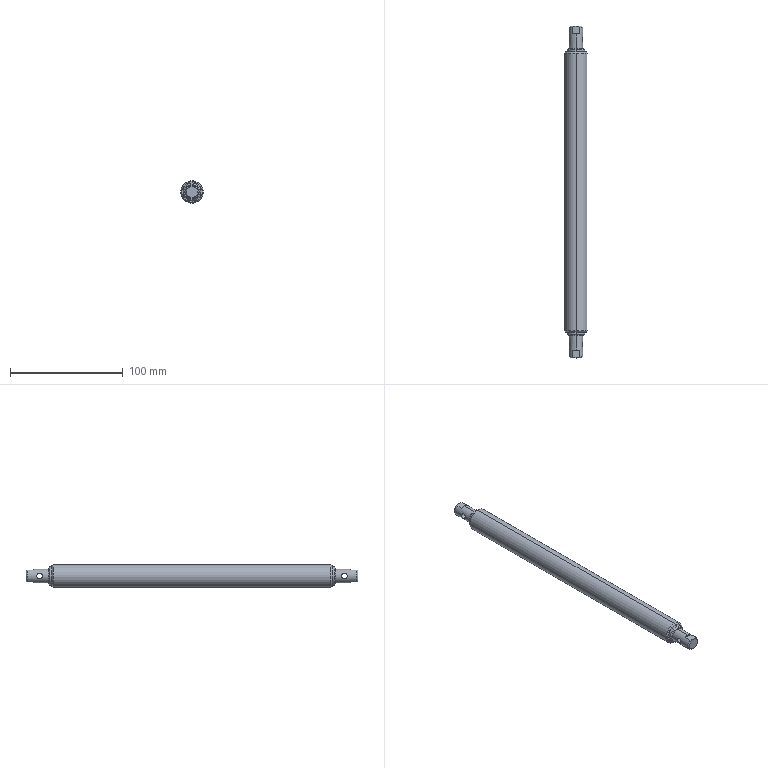Component | SolidWorks | SlideRod-3 | 1 solid | 40 faces | box 20 x 294 x 20 mm | volume 82921 mm3 | cylinder 14 | plane 14 | cone 12 | commonest cylinder face diameters 5 x4 16 x4 12 x4 20 x2
build123d program:
from build123d import *

# Parameters (mm, degrees)
CHAMFER1_SIZE       = 1
CUT_EXTRUDE1_START  = 13
SKETCH2_OUTSIDE_W   = 81.072
SKETCH2_OUTSIDE_H   = 81.072
SKETCH2_OUTSIDE_W_2 = 30.026
SKETCH2_OUTSIDE_H_2 = 10
CUT_EXTRUDE1_DEPTH  = 262.365
SKETCH3_R           = 2.5
CUT_EXTRUDE2_DEPTH  = 148.679


with BuildPart() as part:
    # Sketch1 → Revolve1 (revolve)
    with BuildSketch(Plane.XY, mode=Mode.PRIVATE) as revolve1_sk:
        Polygon((0, -147), (6, -147), (6, -127), (8, -127), (8, -124), (10, -124), (10, 124), (8, 124), (8, 127), (6, 127), (6, 147), (0, 147), align=None)
    revolve(revolve1_sk.sketch.rotate(Axis((0, 0, 0), (0, -1, 0)), 90), axis=Axis((0, 0, 0), (0, -1, 0)))

    # Chamfer1
    chamfer1_edges = [part.edges().sort_by_distance(p)[0] for p in [
        (0, -124, -10),
        (0, 124, -10),
        (0, 127, -8),
        (0, 147, -6),
        (0, -147, -6),
        (0, -127, -8),
    ]]
    chamfer(chamfer1_edges, length=CHAMFER1_SIZE)

    # Sketch2 outside → Cut-Extrude1 (cut, through all)
    with BuildSketch(Plane(origin=(0, 127, 0), x_dir=(1, 0, 0), z_dir=(0, 1, 0)).offset(CUT_EXTRUDE1_START)):
        Rectangle(SKETCH2_OUTSIDE_W, SKETCH2_OUTSIDE_H)
        Rectangle(SKETCH2_OUTSIDE_W_2, SKETCH2_OUTSIDE_H_2, mode=Mode.SUBTRACT)
    cut_extrude1 = extrude(amount=CUT_EXTRUDE1_DEPTH, mode=Mode.SUBTRACT)

    # Sketch3 → Cut-Extrude2 (cut, symmetric)
    with BuildSketch(Plane(origin=(0, 0, 0), x_dir=(0, 0, -1), z_dir=(1, 0, 0))):
        with Locations((0, 135)):
            Circle(SKETCH3_R)
    cut_extrude2 = extrude(amount=CUT_EXTRUDE2_DEPTH, both=True, mode=Mode.SUBTRACT)

    # Mirror1: Cut-Extrude1, Cut-Extrude2 across plane
    add(cut_extrude1.mirror(Plane.ZX), mode=Mode.SUBTRACT)
    add(cut_extrude2.mirror(Plane.ZX), mode=Mode.SUBTRACT)


solid = part.part

# Placed as in the assembly
solid = solid.moved(Location((-261.704, 0, -60), (0, 0, 0)))